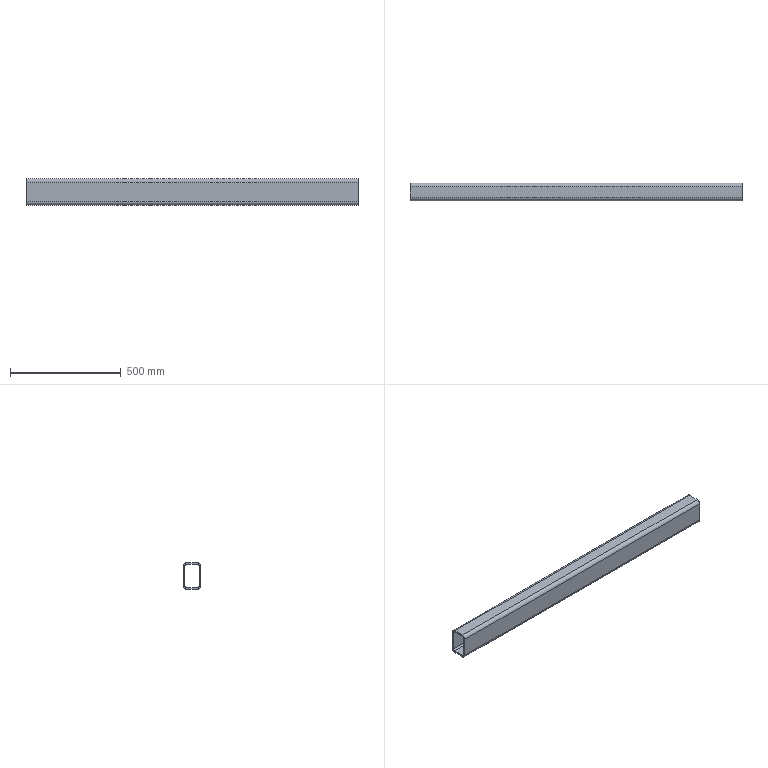Component | SolidWorks | ST60-02-1 | 1 solid | 18 faces | box 1500 x 80 x 120 mm | volume 4168779 mm3 | plane 10 | cylinder 8 | commonest cylinder face diameters 32 x4 16 x4
build123d program:
from build123d import *

# Parameters (mm, degrees)
RECTANGULAR_TUBE_120_X_80_X_8_1_DEPTH = 1500


with BuildPart() as part:
    # Sketch1 → Rectangular Tube 120 X 80 X 8_1 (new body)
    with BuildSketch(Plane.YZ):
        with BuildLine():
            Line((-24, -60), (24, -60))
            ThreePointArc((24, -60), (35.314, -55.314), (40, -44))
            Line((40, -44), (40, 44))
            ThreePointArc((40, 44), (35.314, 55.314), (24, 60))
            Line((24, 60), (-24, 60))
            ThreePointArc((-24, 60), (-35.314, 55.314), (-40, 44))
            Line((-40, 44), (-40, -44))
            ThreePointArc((-40, -44), (-35.314, -55.314), (-24, -60))
        make_face()
        with BuildLine():
            Line((-24, -52), (24, -52))
            ThreePointArc((24, -52), (29.657, -49.657), (32, -44))
            Line((32, -44), (32, 44))
            ThreePointArc((32, 44), (29.657, 49.657), (24, 52))
            Line((24, 52), (-24, 52))
            ThreePointArc((-24, 52), (-29.657, 49.657), (-32, 44))
            Line((-32, 44), (-32, -44))
            ThreePointArc((-32, -44), (-29.657, -49.657), (-24, -52))
        make_face(mode=Mode.SUBTRACT)
    extrude(amount=RECTANGULAR_TUBE_120_X_80_X_8_1_DEPTH)


solid = part.part

# Placed as in the assembly
solid = solid.moved(Location((-847.007, -4.546, 0), (0, 0, 0)))
STEP:
#1=CARTESIAN_POINT('',(-33.347,1.396,1.732));
#2=VERTEX_POINT('',#1);
#3=CARTESIAN_POINT('',(-33.347,0.7659,2.362));
#4=VERTEX_POINT('',#3);
#5=CARTESIAN_POINT('',(-33.347,0.7659,1.732));
#6=DIRECTION('',(1.,0.,0.));
#7=DIRECTION('',(0.,0.,-1.));
#8=AXIS2_PLACEMENT_3D('',#5,#6,#7);
#9=CIRCLE('',#8,0.6299);
#10=EDGE_CURVE('',#2,#4,#9,.T.);
#11=ORIENTED_EDGE('',*,*,#10,.T.);
#12=CARTESIAN_POINT('',(25.708,0.7659,2.362));
#13=VERTEX_POINT('',#12);
#14=CARTESIAN_POINT('',(25.708,0.7659,2.362));
#15=DIRECTION('',(-1.,0.,0.));
#16=VECTOR('',#15,39.37);
#17=LINE('',#14,#16);
#18=EDGE_CURVE('',#13,#4,#17,.T.);
#19=ORIENTED_EDGE('',*,*,#18,.F.);
#20=CARTESIAN_POINT('',(25.708,1.396,1.732));
#21=VERTEX_POINT('',#20);
#22=CARTESIAN_POINT('',(25.708,0.7659,1.732));
#23=DIRECTION('',(1.,0.,0.));
#24=DIRECTION('',(0.,0.,-1.));
#25=AXIS2_PLACEMENT_3D('',#22,#23,#24);
#26=CIRCLE('',#25,0.6299);
#27=EDGE_CURVE('',#21,#13,#26,.T.);
#28=ORIENTED_EDGE('',*,*,#27,.F.);
#29=CARTESIAN_POINT('',(25.708,1.396,1.732));
#30=DIRECTION('',(-1.,0.,0.));
#31=VECTOR('',#30,39.37);
#32=LINE('',#29,#31);
#33=EDGE_CURVE('',#21,#2,#32,.T.);
#34=ORIENTED_EDGE('',*,*,#33,.T.);
#35=EDGE_LOOP('',(#11,#19,#28,#34));
#36=FACE_OUTER_BOUND('',#35,.T.);
#37=CARTESIAN_POINT('',(25.708,0.7659,1.732));
#38=DIRECTION('',(-1.,0.,0.));
#39=DIRECTION('',(0.,0.,1.));
#40=AXIS2_PLACEMENT_3D('',#37,#38,#39);
#41=CYLINDRICAL_SURFACE('',#40,0.6299);
#42=ADVANCED_FACE('',(#36),#41,.T.);
#43=CARTESIAN_POINT('',(-33.347,-1.124,2.362));
#44=VERTEX_POINT('',#43);
#45=CARTESIAN_POINT('',(-33.347,0.7659,2.362));
#46=DIRECTION('',(0.,-1.,0.));
#47=VECTOR('',#46,39.37);
#48=LINE('',#45,#47);
#49=EDGE_CURVE('',#4,#44,#48,.T.);
#50=ORIENTED_EDGE('',*,*,#49,.T.);
#51=CARTESIAN_POINT('',(25.708,-1.124,2.362));
#52=VERTEX_POINT('',#51);
#53=CARTESIAN_POINT('',(25.708,-1.124,2.362));
#54=DIRECTION('',(-1.,0.,0.));
#55=VECTOR('',#54,39.37);
#56=LINE('',#53,#55);
#57=EDGE_CURVE('',#52,#44,#56,.T.);
#58=ORIENTED_EDGE('',*,*,#57,.F.);
#59=CARTESIAN_POINT('',(25.708,0.7659,2.362));
#60=DIRECTION('',(0.,-1.,0.));
#61=VECTOR('',#60,39.37);
#62=LINE('',#59,#61);
#63=EDGE_CURVE('',#13,#52,#62,.T.);
#64=ORIENTED_EDGE('',*,*,#63,.F.);
#65=ORIENTED_EDGE('',*,*,#18,.T.);
#66=EDGE_LOOP('',(#50,#58,#64,#65));
#67=FACE_OUTER_BOUND('',#66,.T.);
#68=CARTESIAN_POINT('',(25.708,0.7659,2.362));
#69=DIRECTION('',(0.,0.,-1.));
#70=DIRECTION('',(-1.,0.,0.));
#71=AXIS2_PLACEMENT_3D('',#68,#69,#70);
#72=PLANE('',#71);
#73=ADVANCED_FACE('',(#67),#72,.F.);
#74=CARTESIAN_POINT('',(-33.347,-1.754,1.732));
#75=VERTEX_POINT('',#74);
#76=CARTESIAN_POINT('',(-33.347,-1.124,1.732));
#77=DIRECTION('',(1.,0.,0.));
#78=DIRECTION('',(0.,0.,-1.));
#79=AXIS2_PLACEMENT_3D('',#76,#77,#78);
#80=CIRCLE('',#79,0.6299);
#81=EDGE_CURVE('',#44,#75,#80,.T.);
#82=ORIENTED_EDGE('',*,*,#81,.T.);
#83=CARTESIAN_POINT('',(25.708,-1.754,1.732));
#84=VERTEX_POINT('',#83);
#85=CARTESIAN_POINT('',(25.708,-1.754,1.732));
#86=DIRECTION('',(-1.,0.,0.));
#87=VECTOR('',#86,39.37);
#88=LINE('',#85,#87);
#89=EDGE_CURVE('',#84,#75,#88,.T.);
#90=ORIENTED_EDGE('',*,*,#89,.F.);
#91=CARTESIAN_POINT('',(25.708,-1.124,1.732));
#92=DIRECTION('',(1.,0.,0.));
#93=DIRECTION('',(0.,0.,-1.));
#94=AXIS2_PLACEMENT_3D('',#91,#92,#93);
#95=CIRCLE('',#94,0.6299);
#96=EDGE_CURVE('',#52,#84,#95,.T.);
#97=ORIENTED_EDGE('',*,*,#96,.F.);
#98=ORIENTED_EDGE('',*,*,#57,.T.);
#99=EDGE_LOOP('',(#82,#90,#97,#98));
#100=FACE_OUTER_BOUND('',#99,.T.);
#101=CARTESIAN_POINT('',(25.708,-1.124,1.732));
#102=DIRECTION('',(-1.,0.,0.));
#103=DIRECTION('',(0.,0.,1.));
#104=AXIS2_PLACEMENT_3D('',#101,#102,#103);
#105=CYLINDRICAL_SURFACE('',#104,0.6299);
#106=ADVANCED_FACE('',(#100),#105,.T.);
#107=CARTESIAN_POINT('',(-33.347,-1.754,-1.732));
#108=VERTEX_POINT('',#107);
#109=CARTESIAN_POINT('',(-33.347,-1.754,-1.732));
#110=DIRECTION('',(0.,0.,-1.));
#111=VECTOR('',#110,39.37);
#112=LINE('',#109,#111);
#113=EDGE_CURVE('',#75,#108,#112,.T.);
#114=ORIENTED_EDGE('',*,*,#113,.T.);
#115=CARTESIAN_POINT('',(25.708,-1.754,-1.732));
#116=VERTEX_POINT('',#115);
#117=CARTESIAN_POINT('',(25.708,-1.754,-1.732));
#118=DIRECTION('',(-1.,0.,0.));
#119=VECTOR('',#118,39.37);
#120=LINE('',#117,#119);
#121=EDGE_CURVE('',#116,#108,#120,.T.);
#122=ORIENTED_EDGE('',*,*,#121,.F.);
#123=CARTESIAN_POINT('',(25.708,-1.754,-1.732));
#124=DIRECTION('',(0.,0.,-1.));
#125=VECTOR('',#124,39.37);
#126=LINE('',#123,#125);
#127=EDGE_CURVE('',#84,#116,#126,.T.);
#128=ORIENTED_EDGE('',*,*,#127,.F.);
#129=ORIENTED_EDGE('',*,*,#89,.T.);
#130=EDGE_LOOP('',(#114,#122,#128,#129));
#131=FACE_OUTER_BOUND('',#130,.T.);
#132=CARTESIAN_POINT('',(25.708,-1.754,-1.732));
#133=DIRECTION('',(0.,1.,0.));
#134=DIRECTION('',(0.,0.,1.));
#135=AXIS2_PLACEMENT_3D('',#132,#133,#134);
#136=PLANE('',#135);
#137=ADVANCED_FACE('',(#131),#136,.F.);
#138=CARTESIAN_POINT('',(-33.347,-1.124,-2.362));
#139=VERTEX_POINT('',#138);
#140=CARTESIAN_POINT('',(-33.347,-1.124,-1.732));
#141=DIRECTION('',(1.,0.,0.));
#142=DIRECTION('',(0.,0.,-1.));
#143=AXIS2_PLACEMENT_3D('',#140,#141,#142);
#144=CIRCLE('',#143,0.6299);
#145=EDGE_CURVE('',#108,#139,#144,.T.);
#146=ORIENTED_EDGE('',*,*,#145,.T.);
#147=CARTESIAN_POINT('',(25.708,-1.124,-2.362));
#148=VERTEX_POINT('',#147);
#149=CARTESIAN_POINT('',(25.708,-1.124,-2.362));
#150=DIRECTION('',(-1.,0.,0.));
#151=VECTOR('',#150,39.37);
#152=LINE('',#149,#151);
#153=EDGE_CURVE('',#148,#139,#152,.T.);
#154=ORIENTED_EDGE('',*,*,#153,.F.);
#155=CARTESIAN_POINT('',(25.708,-1.124,-1.732));
#156=DIRECTION('',(1.,0.,0.));
#157=DIRECTION('',(0.,0.,-1.));
#158=AXIS2_PLACEMENT_3D('',#155,#156,#157);
#159=CIRCLE('',#158,0.6299);
#160=EDGE_CURVE('',#116,#148,#159,.T.);
#161=ORIENTED_EDGE('',*,*,#160,.F.);
#162=ORIENTED_EDGE('',*,*,#121,.T.);
#163=EDGE_LOOP('',(#146,#154,#161,#162));
#164=FACE_OUTER_BOUND('',#163,.T.);
#165=CARTESIAN_POINT('',(25.708,-1.124,-1.732));
#166=DIRECTION('',(-1.,0.,0.));
#167=DIRECTION('',(0.,0.,1.));
#168=AXIS2_PLACEMENT_3D('',#165,#166,#167);
#169=CYLINDRICAL_SURFACE('',#168,0.6299);
#170=ADVANCED_FACE('',(#164),#169,.T.);
#171=CARTESIAN_POINT('',(-33.347,0.7659,-2.362));
#172=VERTEX_POINT('',#171);
#173=CARTESIAN_POINT('',(-33.347,-1.124,-2.362));
#174=DIRECTION('',(0.,1.,0.));
#175=VECTOR('',#174,39.37);
#176=LINE('',#173,#175);
#177=EDGE_CURVE('',#139,#172,#176,.T.);
#178=ORIENTED_EDGE('',*,*,#177,.T.);
#179=CARTESIAN_POINT('',(25.708,0.7659,-2.362));
#180=VERTEX_POINT('',#179);
#181=CARTESIAN_POINT('',(25.708,0.7659,-2.362));
#182=DIRECTION('',(-1.,0.,0.));
#183=VECTOR('',#182,39.37);
#184=LINE('',#181,#183);
#185=EDGE_CURVE('',#180,#172,#184,.T.);
#186=ORIENTED_EDGE('',*,*,#185,.F.);
#187=CARTESIAN_POINT('',(25.708,-1.124,-2.362));
#188=DIRECTION('',(0.,1.,0.));
#189=VECTOR('',#188,39.37);
#190=LINE('',#187,#189);
#191=EDGE_CURVE('',#148,#180,#190,.T.);
#192=ORIENTED_EDGE('',*,*,#191,.F.);
#193=ORIENTED_EDGE('',*,*,#153,.T.);
#194=EDGE_LOOP('',(#178,#186,#192,#193));
#195=FACE_OUTER_BOUND('',#194,.T.);
#196=CARTESIAN_POINT('',(25.708,-1.124,-2.362));
#197=DIRECTION('',(0.,0.,1.));
#198=DIRECTION('',(1.,0.,0.));
#199=AXIS2_PLACEMENT_3D('',#196,#197,#198);
#200=PLANE('',#199);
#201=ADVANCED_FACE('',(#195),#200,.F.);
#202=CARTESIAN_POINT('',(-33.347,1.396,-1.732));
#203=VERTEX_POINT('',#202);
#204=CARTESIAN_POINT('',(-33.347,0.7659,-1.732));
#205=DIRECTION('',(1.,0.,0.));
#206=DIRECTION('',(0.,0.,-1.));
#207=AXIS2_PLACEMENT_3D('',#204,#205,#206);
#208=CIRCLE('',#207,0.6299);
#209=EDGE_CURVE('',#172,#203,#208,.T.);
#210=ORIENTED_EDGE('',*,*,#209,.T.);
#211=CARTESIAN_POINT('',(25.708,1.396,-1.732));
#212=VERTEX_POINT('',#211);
#213=CARTESIAN_POINT('',(25.708,1.396,-1.732));
#214=DIRECTION('',(-1.,0.,0.));
#215=VECTOR('',#214,39.37);
#216=LINE('',#213,#215);
#217=EDGE_CURVE('',#212,#203,#216,.T.);
#218=ORIENTED_EDGE('',*,*,#217,.F.);
#219=CARTESIAN_POINT('',(25.708,0.7659,-1.732));
#220=DIRECTION('',(1.,0.,0.));
#221=DIRECTION('',(0.,0.,-1.));
#222=AXIS2_PLACEMENT_3D('',#219,#220,#221);
#223=CIRCLE('',#222,0.6299);
#224=EDGE_CURVE('',#180,#212,#223,.T.);
#225=ORIENTED_EDGE('',*,*,#224,.F.);
#226=ORIENTED_EDGE('',*,*,#185,.T.);
#227=EDGE_LOOP('',(#210,#218,#225,#226));
#228=FACE_OUTER_BOUND('',#227,.T.);
#229=CARTESIAN_POINT('',(25.708,0.7659,-1.732));
#230=DIRECTION('',(-1.,0.,0.));
#231=DIRECTION('',(0.,0.,1.));
#232=AXIS2_PLACEMENT_3D('',#229,#230,#231);
#233=CYLINDRICAL_SURFACE('',#232,0.6299);
#234=ADVANCED_FACE('',(#228),#233,.T.);
#235=CARTESIAN_POINT('',(-33.347,-1.124,2.047));
#236=VERTEX_POINT('',#235);
#237=CARTESIAN_POINT('',(-33.347,-1.439,1.732));
#238=VERTEX_POINT('',#237);
#239=CARTESIAN_POINT('',(-33.347,-1.124,1.732));
#240=DIRECTION('',(1.,0.,0.));
#241=DIRECTION('',(0.,0.,-1.));
#242=AXIS2_PLACEMENT_3D('',#239,#240,#241);
#243=CIRCLE('',#242,0.315);
#244=EDGE_CURVE('',#236,#238,#243,.T.);
#245=ORIENTED_EDGE('',*,*,#244,.F.);
#246=CARTESIAN_POINT('',(25.708,-1.124,2.047));
#247=VERTEX_POINT('',#246);
#248=CARTESIAN_POINT('',(25.708,-1.124,2.047));
#249=DIRECTION('',(-1.,0.,0.));
#250=VECTOR('',#249,39.37);
#251=LINE('',#248,#250);
#252=EDGE_CURVE('',#247,#236,#251,.T.);
#253=ORIENTED_EDGE('',*,*,#252,.F.);
#254=CARTESIAN_POINT('',(25.708,-1.439,1.732));
#255=VERTEX_POINT('',#254);
#256=CARTESIAN_POINT('',(25.708,-1.124,1.732));
#257=DIRECTION('',(1.,0.,0.));
#258=DIRECTION('',(0.,0.,-1.));
#259=AXIS2_PLACEMENT_3D('',#256,#257,#258);
#260=CIRCLE('',#259,0.315);
#261=EDGE_CURVE('',#247,#255,#260,.T.);
#262=ORIENTED_EDGE('',*,*,#261,.T.);
#263=CARTESIAN_POINT('',(25.708,-1.439,1.732));
#264=DIRECTION('',(-1.,0.,0.));
#265=VECTOR('',#264,39.37);
#266=LINE('',#263,#265);
#267=EDGE_CURVE('',#255,#238,#266,.T.);
#268=ORIENTED_EDGE('',*,*,#267,.T.);
#269=EDGE_LOOP('',(#245,#253,#262,#268));
#270=FACE_OUTER_BOUND('',#269,.T.);
#271=CARTESIAN_POINT('',(25.708,-1.124,1.732));
#272=DIRECTION('',(-1.,0.,0.));
#273=DIRECTION('',(0.,0.,1.));
#274=AXIS2_PLACEMENT_3D('',#271,#272,#273);
#275=CYLINDRICAL_SURFACE('',#274,0.315);
#276=ADVANCED_FACE('',(#270),#275,.F.);
#277=CARTESIAN_POINT('',(-33.347,0.7659,2.047));
#278=VERTEX_POINT('',#277);
#279=CARTESIAN_POINT('',(-33.347,0.7659,2.047));
#280=DIRECTION('',(0.,-1.,0.));
#281=VECTOR('',#280,39.37);
#282=LINE('',#279,#281);
#283=EDGE_CURVE('',#278,#236,#282,.T.);
#284=ORIENTED_EDGE('',*,*,#283,.F.);
#285=CARTESIAN_POINT('',(25.708,0.7659,2.047));
#286=VERTEX_POINT('',#285);
#287=CARTESIAN_POINT('',(25.708,0.7659,2.047));
#288=DIRECTION('',(-1.,0.,0.));
#289=VECTOR('',#288,39.37);
#290=LINE('',#287,#289);
#291=EDGE_CURVE('',#286,#278,#290,.T.);
#292=ORIENTED_EDGE('',*,*,#291,.F.);
#293=CARTESIAN_POINT('',(25.708,0.7659,2.047));
#294=DIRECTION('',(0.,-1.,0.));
#295=VECTOR('',#294,39.37);
#296=LINE('',#293,#295);
#297=EDGE_CURVE('',#286,#247,#296,.T.);
#298=ORIENTED_EDGE('',*,*,#297,.T.);
#299=ORIENTED_EDGE('',*,*,#252,.T.);
#300=EDGE_LOOP('',(#284,#292,#298,#299));
#301=FACE_OUTER_BOUND('',#300,.T.);
#302=CARTESIAN_POINT('',(25.708,0.7659,2.047));
#303=DIRECTION('',(0.,0.,-1.));
#304=DIRECTION('',(-1.,0.,0.));
#305=AXIS2_PLACEMENT_3D('',#302,#303,#304);
#306=PLANE('',#305);
#307=ADVANCED_FACE('',(#301),#306,.T.);
#308=CARTESIAN_POINT('',(-33.347,1.081,1.732));
#309=VERTEX_POINT('',#308);
#310=CARTESIAN_POINT('',(-33.347,0.7659,1.732));
#311=DIRECTION('',(1.,0.,0.));
#312=DIRECTION('',(0.,0.,-1.));
#313=AXIS2_PLACEMENT_3D('',#310,#311,#312);
#314=CIRCLE('',#313,0.315);
#315=EDGE_CURVE('',#309,#278,#314,.T.);
#316=ORIENTED_EDGE('',*,*,#315,.F.);
#317=CARTESIAN_POINT('',(25.708,1.081,1.732));
#318=VERTEX_POINT('',#317);
#319=CARTESIAN_POINT('',(25.708,1.081,1.732));
#320=DIRECTION('',(-1.,0.,0.));
#321=VECTOR('',#320,39.37);
#322=LINE('',#319,#321);
#323=EDGE_CURVE('',#318,#309,#322,.T.);
#324=ORIENTED_EDGE('',*,*,#323,.F.);
#325=CARTESIAN_POINT('',(25.708,0.7659,1.732));
#326=DIRECTION('',(1.,0.,0.));
#327=DIRECTION('',(0.,0.,-1.));
#328=AXIS2_PLACEMENT_3D('',#325,#326,#327);
#329=CIRCLE('',#328,0.315);
#330=EDGE_CURVE('',#318,#286,#329,.T.);
#331=ORIENTED_EDGE('',*,*,#330,.T.);
#332=ORIENTED_EDGE('',*,*,#291,.T.);
#333=EDGE_LOOP('',(#316,#324,#331,#332));
#334=FACE_OUTER_BOUND('',#333,.T.);
#335=CARTESIAN_POINT('',(25.708,0.7659,1.732));
#336=DIRECTION('',(-1.,0.,0.));
#337=DIRECTION('',(0.,0.,1.));
#338=AXIS2_PLACEMENT_3D('',#335,#336,#337);
#339=CYLINDRICAL_SURFACE('',#338,0.315);
#340=ADVANCED_FACE('',(#334),#339,.F.);
#341=CARTESIAN_POINT('',(-33.347,1.081,-1.732));
#342=VERTEX_POINT('',#341);
#343=CARTESIAN_POINT('',(-33.347,1.081,1.732));
#344=DIRECTION('',(0.,0.,1.));
#345=VECTOR('',#344,39.37);
#346=LINE('',#343,#345);
#347=EDGE_CURVE('',#342,#309,#346,.T.);
#348=ORIENTED_EDGE('',*,*,#347,.F.);
#349=CARTESIAN_POINT('',(25.708,1.081,-1.732));
#350=VERTEX_POINT('',#349);
#351=CARTESIAN_POINT('',(25.708,1.081,-1.732));
#352=DIRECTION('',(-1.,0.,0.));
#353=VECTOR('',#352,39.37);
#354=LINE('',#351,#353);
#355=EDGE_CURVE('',#350,#342,#354,.T.);
#356=ORIENTED_EDGE('',*,*,#355,.F.);
#357=CARTESIAN_POINT('',(25.708,1.081,1.732));
#358=DIRECTION('',(0.,0.,1.));
#359=VECTOR('',#358,39.37);
#360=LINE('',#357,#359);
#361=EDGE_CURVE('',#350,#318,#360,.T.);
#362=ORIENTED_EDGE('',*,*,#361,.T.);
#363=ORIENTED_EDGE('',*,*,#323,.T.);
#364=EDGE_LOOP('',(#348,#356,#362,#363));
#365=FACE_OUTER_BOUND('',#364,.T.);
#366=CARTESIAN_POINT('',(25.708,1.081,1.732));
#367=DIRECTION('',(0.,-1.,0.));
#368=DIRECTION('',(0.,0.,-1.));
#369=AXIS2_PLACEMENT_3D('',#366,#367,#368);
#370=PLANE('',#369);
#371=ADVANCED_FACE('',(#365),#370,.T.);
#372=CARTESIAN_POINT('',(-33.347,0.7659,-2.047));
#373=VERTEX_POINT('',#372);
#374=CARTESIAN_POINT('',(-33.347,0.7659,-1.732));
#375=DIRECTION('',(1.,0.,0.));
#376=DIRECTION('',(0.,0.,-1.));
#377=AXIS2_PLACEMENT_3D('',#374,#375,#376);
#378=CIRCLE('',#377,0.315);
#379=EDGE_CURVE('',#373,#342,#378,.T.);
#380=ORIENTED_EDGE('',*,*,#379,.F.);
#381=CARTESIAN_POINT('',(25.708,0.7659,-2.047));
#382=VERTEX_POINT('',#381);
#383=CARTESIAN_POINT('',(25.708,0.7659,-2.047));
#384=DIRECTION('',(-1.,0.,0.));
#385=VECTOR('',#384,39.37);
#386=LINE('',#383,#385);
#387=EDGE_CURVE('',#382,#373,#386,.T.);
#388=ORIENTED_EDGE('',*,*,#387,.F.);
#389=CARTESIAN_POINT('',(25.708,0.7659,-1.732));
#390=DIRECTION('',(1.,0.,0.));
#391=DIRECTION('',(0.,0.,-1.));
#392=AXIS2_PLACEMENT_3D('',#389,#390,#391);
#393=CIRCLE('',#392,0.315);
#394=EDGE_CURVE('',#382,#350,#393,.T.);
#395=ORIENTED_EDGE('',*,*,#394,.T.);
#396=ORIENTED_EDGE('',*,*,#355,.T.);
#397=EDGE_LOOP('',(#380,#388,#395,#396));
#398=FACE_OUTER_BOUND('',#397,.T.);
#399=CARTESIAN_POINT('',(25.708,0.7659,-1.732));
#400=DIRECTION('',(-1.,0.,0.));
#401=DIRECTION('',(0.,0.,1.));
#402=AXIS2_PLACEMENT_3D('',#399,#400,#401);
#403=CYLINDRICAL_SURFACE('',#402,0.315);
#404=ADVANCED_FACE('',(#398),#403,.F.);
#405=CARTESIAN_POINT('',(-33.347,-1.124,-2.047));
#406=VERTEX_POINT('',#405);
#407=CARTESIAN_POINT('',(-33.347,-1.124,-2.047));
#408=DIRECTION('',(0.,1.,0.));
#409=VECTOR('',#408,39.37);
#410=LINE('',#407,#409);
#411=EDGE_CURVE('',#406,#373,#410,.T.);
#412=ORIENTED_EDGE('',*,*,#411,.F.);
#413=CARTESIAN_POINT('',(25.708,-1.124,-2.047));
#414=VERTEX_POINT('',#413);
#415=CARTESIAN_POINT('',(25.708,-1.124,-2.047));
#416=DIRECTION('',(-1.,0.,0.));
#417=VECTOR('',#416,39.37);
#418=LINE('',#415,#417);
#419=EDGE_CURVE('',#414,#406,#418,.T.);
#420=ORIENTED_EDGE('',*,*,#419,.F.);
#421=CARTESIAN_POINT('',(25.708,-1.124,-2.047));
#422=DIRECTION('',(0.,1.,0.));
#423=VECTOR('',#422,39.37);
#424=LINE('',#421,#423);
#425=EDGE_CURVE('',#414,#382,#424,.T.);
#426=ORIENTED_EDGE('',*,*,#425,.T.);
#427=ORIENTED_EDGE('',*,*,#387,.T.);
#428=EDGE_LOOP('',(#412,#420,#426,#427));
#429=FACE_OUTER_BOUND('',#428,.T.);
#430=CARTESIAN_POINT('',(25.708,-1.124,-2.047));
#431=DIRECTION('',(0.,0.,1.));
#432=DIRECTION('',(1.,0.,0.));
#433=AXIS2_PLACEMENT_3D('',#430,#431,#432);
#434=PLANE('',#433);
#435=ADVANCED_FACE('',(#429),#434,.T.);
#436=CARTESIAN_POINT('',(-33.347,-1.439,-1.732));
#437=VERTEX_POINT('',#436);
#438=CARTESIAN_POINT('',(-33.347,-1.124,-1.732));
#439=DIRECTION('',(1.,0.,0.));
#440=DIRECTION('',(0.,0.,-1.));
#441=AXIS2_PLACEMENT_3D('',#438,#439,#440);
#442=CIRCLE('',#441,0.315);
#443=EDGE_CURVE('',#437,#406,#442,.T.);
#444=ORIENTED_EDGE('',*,*,#443,.F.);
#445=CARTESIAN_POINT('',(25.708,-1.439,-1.732));
#446=VERTEX_POINT('',#445);
#447=CARTESIAN_POINT('',(25.708,-1.439,-1.732));
#448=DIRECTION('',(-1.,0.,0.));
#449=VECTOR('',#448,39.37);
#450=LINE('',#447,#449);
#451=EDGE_CURVE('',#446,#437,#450,.T.);
#452=ORIENTED_EDGE('',*,*,#451,.F.);
#453=CARTESIAN_POINT('',(25.708,-1.124,-1.732));
#454=DIRECTION('',(1.,0.,0.));
#455=DIRECTION('',(0.,0.,-1.));
#456=AXIS2_PLACEMENT_3D('',#453,#454,#455);
#457=CIRCLE('',#456,0.315);
#458=EDGE_CURVE('',#446,#414,#457,.T.);
#459=ORIENTED_EDGE('',*,*,#458,.T.);
#460=ORIENTED_EDGE('',*,*,#419,.T.);
#461=EDGE_LOOP('',(#444,#452,#459,#460));
#462=FACE_OUTER_BOUND('',#461,.T.);
#463=CARTESIAN_POINT('',(25.708,-1.124,-1.732));
#464=DIRECTION('',(-1.,0.,0.));
#465=DIRECTION('',(0.,0.,1.));
#466=AXIS2_PLACEMENT_3D('',#463,#464,#465);
#467=CYLINDRICAL_SURFACE('',#466,0.315);
#468=ADVANCED_FACE('',(#462),#467,.F.);
#469=CARTESIAN_POINT('',(-33.347,-1.439,-1.732));
#470=DIRECTION('',(0.,0.,-1.));
#471=VECTOR('',#470,39.37);
#472=LINE('',#469,#471);
#473=EDGE_CURVE('',#238,#437,#472,.T.);
#474=ORIENTED_EDGE('',*,*,#473,.F.);
#475=ORIENTED_EDGE('',*,*,#267,.F.);
#476=CARTESIAN_POINT('',(25.708,-1.439,-1.732));
#477=DIRECTION('',(0.,0.,-1.));
#478=VECTOR('',#477,39.37);
#479=LINE('',#476,#478);
#480=EDGE_CURVE('',#255,#446,#479,.T.);
#481=ORIENTED_EDGE('',*,*,#480,.T.);
#482=ORIENTED_EDGE('',*,*,#451,.T.);
#483=EDGE_LOOP('',(#474,#475,#481,#482));
#484=FACE_OUTER_BOUND('',#483,.T.);
#485=CARTESIAN_POINT('',(25.708,-1.439,-1.732));
#486=DIRECTION('',(0.,1.,0.));
#487=DIRECTION('',(0.,0.,1.));
#488=AXIS2_PLACEMENT_3D('',#485,#486,#487);
#489=PLANE('',#488);
#490=ADVANCED_FACE('',(#484),#489,.T.);
#491=CARTESIAN_POINT('',(-33.347,1.396,1.732));
#492=DIRECTION('',(0.,0.,1.));
#493=VECTOR('',#492,39.37);
#494=LINE('',#491,#493);
#495=EDGE_CURVE('',#203,#2,#494,.T.);
#496=ORIENTED_EDGE('',*,*,#495,.T.);
#497=ORIENTED_EDGE('',*,*,#33,.F.);
#498=CARTESIAN_POINT('',(25.708,1.396,1.732));
#499=DIRECTION('',(0.,0.,1.));
#500=VECTOR('',#499,39.37);
#501=LINE('',#498,#500);
#502=EDGE_CURVE('',#212,#21,#501,.T.);
#503=ORIENTED_EDGE('',*,*,#502,.F.);
#504=ORIENTED_EDGE('',*,*,#217,.T.);
#505=EDGE_LOOP('',(#496,#497,#503,#504));
#506=FACE_OUTER_BOUND('',#505,.T.);
#507=CARTESIAN_POINT('',(25.708,1.396,1.732));
#508=DIRECTION('',(0.,-1.,0.));
#509=DIRECTION('',(0.,0.,-1.));
#510=AXIS2_PLACEMENT_3D('',#507,#508,#509);
#511=PLANE('',#510);
#512=ADVANCED_FACE('',(#506),#511,.F.);
#513=ORIENTED_EDGE('',*,*,#261,.F.);
#514=ORIENTED_EDGE('',*,*,#297,.F.);
#515=ORIENTED_EDGE('',*,*,#330,.F.);
#516=ORIENTED_EDGE('',*,*,#361,.F.);
#517=ORIENTED_EDGE('',*,*,#394,.F.);
#518=ORIENTED_EDGE('',*,*,#425,.F.);
#519=ORIENTED_EDGE('',*,*,#458,.F.);
#520=ORIENTED_EDGE('',*,*,#480,.F.);
#521=EDGE_LOOP('',(#513,#514,#515,#516,#517,#518,#519,#520));
#522=FACE_BOUND('',#521,.T.);
#523=ORIENTED_EDGE('',*,*,#27,.T.);
#524=ORIENTED_EDGE('',*,*,#63,.T.);
#525=ORIENTED_EDGE('',*,*,#96,.T.);
#526=ORIENTED_EDGE('',*,*,#127,.T.);
#527=ORIENTED_EDGE('',*,*,#160,.T.);
#528=ORIENTED_EDGE('',*,*,#191,.T.);
#529=ORIENTED_EDGE('',*,*,#224,.T.);
#530=ORIENTED_EDGE('',*,*,#502,.T.);
#531=EDGE_LOOP('',(#523,#524,#525,#526,#527,#528,#529,#530));
#532=FACE_OUTER_BOUND('',#531,.T.);
#533=CARTESIAN_POINT('',(25.708,0.7659,1.732));
#534=DIRECTION('',(1.,0.,0.));
#535=DIRECTION('',(0.,0.,-1.));
#536=AXIS2_PLACEMENT_3D('',#533,#534,#535);
#537=PLANE('',#536);
#538=ADVANCED_FACE('',(#522,#532),#537,.T.);
#539=ORIENTED_EDGE('',*,*,#244,.T.);
#540=ORIENTED_EDGE('',*,*,#473,.T.);
#541=ORIENTED_EDGE('',*,*,#443,.T.);
#542=ORIENTED_EDGE('',*,*,#411,.T.);
#543=ORIENTED_EDGE('',*,*,#379,.T.);
#544=ORIENTED_EDGE('',*,*,#347,.T.);
#545=ORIENTED_EDGE('',*,*,#315,.T.);
#546=ORIENTED_EDGE('',*,*,#283,.T.);
#547=EDGE_LOOP('',(#539,#540,#541,#542,#543,#544,#545,#546));
#548=FACE_BOUND('',#547,.T.);
#549=ORIENTED_EDGE('',*,*,#10,.F.);
#550=ORIENTED_EDGE('',*,*,#495,.F.);
#551=ORIENTED_EDGE('',*,*,#209,.F.);
#552=ORIENTED_EDGE('',*,*,#177,.F.);
#553=ORIENTED_EDGE('',*,*,#145,.F.);
#554=ORIENTED_EDGE('',*,*,#113,.F.);
#555=ORIENTED_EDGE('',*,*,#81,.F.);
#556=ORIENTED_EDGE('',*,*,#49,.F.);
#557=EDGE_LOOP('',(#549,#550,#551,#552,#553,#554,#555,#556));
#558=FACE_OUTER_BOUND('',#557,.T.);
#559=CARTESIAN_POINT('',(-33.347,0.7659,1.732));
#560=DIRECTION('',(1.,0.,0.));
#561=DIRECTION('',(0.,0.,-1.));
#562=AXIS2_PLACEMENT_3D('',#559,#560,#561);
#563=PLANE('',#562);
#564=ADVANCED_FACE('',(#548,#558),#563,.F.);
#565=CLOSED_SHELL('',(#42,#73,#106,#137,#170,#201,#234,#276,#307,#340,#371,#404,#435,#468,#490,#512,#538,#564));
#566=MANIFOLD_SOLID_BREP('',#565);
#567=CARTESIAN_POINT('',(0.,0.,0.));
#568=DIRECTION('',(0.,0.,1.));
#569=DIRECTION('',(1.,0.,0.));
#570=AXIS2_PLACEMENT_3D('',#567,#568,#569);
#571=(LENGTH_UNIT()NAMED_UNIT(*)SI_UNIT($,.METRE.));
#572=LENGTH_MEASURE_WITH_UNIT(LENGTH_MEASURE(0.0254),#571);
#573=DIMENSIONAL_EXPONENTS(1.,0.,0.,0.,0.,0.,0.);
#574=(CONVERSION_BASED_UNIT('',#572)LENGTH_UNIT()NAMED_UNIT(#573));
#575=UNCERTAINTY_MEASURE_WITH_UNIT(LENGTH_MEASURE(0.00001),#574,'','');
#576=(NAMED_UNIT(*)PLANE_ANGLE_UNIT()SI_UNIT($,.RADIAN.));
#577=(NAMED_UNIT(*)SI_UNIT($,.STERADIAN.)SOLID_ANGLE_UNIT());
#578=(GEOMETRIC_REPRESENTATION_CONTEXT(3)GLOBAL_UNCERTAINTY_ASSIGNED_CONTEXT((#575))GLOBAL_UNIT_ASSIGNED_CONTEXT((#574,#576,#577))REPRESENTATION_CONTEXT('',''));
#579=ADVANCED_BREP_SHAPE_REPRESENTATION('',(#566,#570),#578);
#580=COLOUR_RGB('',0.7922,0.8196,0.9333);
#581=FILL_AREA_STYLE_COLOUR('',#580);
#582=FILL_AREA_STYLE('',(#581));
#583=SURFACE_STYLE_FILL_AREA(#582);
#584=SURFACE_SIDE_STYLE('',(#583));
#585=SURFACE_STYLE_USAGE(.BOTH.,#584);
#586=PRESENTATION_STYLE_ASSIGNMENT((#585));
#587=STYLED_ITEM('',(#586),#566);
#588=PRESENTATION_LAYER_ASSIGNMENT('','',(#587));
#589=(LENGTH_UNIT()NAMED_UNIT(*)SI_UNIT($,.METRE.));
#590=LENGTH_MEASURE_WITH_UNIT(LENGTH_MEASURE(0.0254),#589);
#591=DIMENSIONAL_EXPONENTS(1.,0.,0.,0.,0.,0.,0.);
#592=(CONVERSION_BASED_UNIT('',#590)LENGTH_UNIT()NAMED_UNIT(#591));
#593=UNCERTAINTY_MEASURE_WITH_UNIT(LENGTH_MEASURE(0.00001),#592,'','');
#594=(NAMED_UNIT(*)PLANE_ANGLE_UNIT()SI_UNIT($,.RADIAN.));
#595=(NAMED_UNIT(*)SI_UNIT($,.STERADIAN.)SOLID_ANGLE_UNIT());
#596=(GEOMETRIC_REPRESENTATION_CONTEXT(3)GLOBAL_UNCERTAINTY_ASSIGNED_CONTEXT((#593))GLOBAL_UNIT_ASSIGNED_CONTEXT((#592,#594,#595))REPRESENTATION_CONTEXT('',''));
#597=MECHANICAL_DESIGN_GEOMETRIC_PRESENTATION_REPRESENTATION('',(#587),#596);